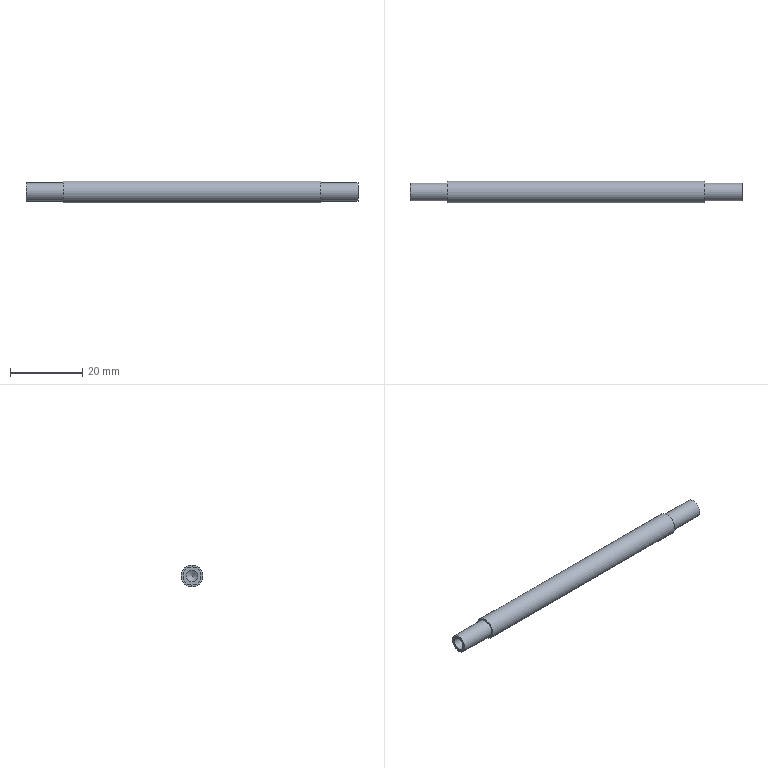Component | NX | WHEEL_AXLE | 1 solid | 11 faces | box 91.6 x 6 x 6 mm | volume 2235 mm3 | cylinder 5 | plane 4 | cone 2 | commonest cylinder face diameters 5 x2 3.3 x2 6 x1
STEP:
#1=CARTESIAN_POINT('',(0.,0.,0.));
#2=DIRECTION('',(0.,0.,1.));
#3=DIRECTION('',(1.,0.,0.));
#4=AXIS2_PLACEMENT_3D('',#1,#2,#3);
#5=CARTESIAN_POINT('',(-49.856,16.19,-74.915));
#6=VERTEX_POINT('',#5);
#7=CARTESIAN_POINT('',(-49.856,16.19,-77.415));
#8=DIRECTION('',(-1.,0.,0.));
#9=DIRECTION('',(0.,0.,1.));
#10=AXIS2_PLACEMENT_3D('',#7,#8,#9);
#11=CIRCLE('',#10,2.5);
#12=CARTESIAN_POINT('',(-60.156,16.19,-77.415));
#13=DIRECTION('',(1.,0.,0.));
#14=DIRECTION('',(0.,0.,-1.));
#15=AXIS2_PLACEMENT_3D('',#12,#13,#14);
#16=CYLINDRICAL_SURFACE('',#15,2.5);
#17=CARTESIAN_POINT('',(9.425,10.3));
#18=DIRECTION('',(-1.,0.));
#19=VECTOR('',#18,1.);
#20=LINE('',#17,#19);
#21=(GEOMETRIC_REPRESENTATION_CONTEXT(2)PARAMETRIC_REPRESENTATION_CONTEXT()REPRESENTATION_CONTEXT('',''));
#22=DEFINITIONAL_REPRESENTATION('',(#20),#21);
#23=PCURVE('',#16,#22);
#24=CARTESIAN_POINT('',(-49.856,16.19,-77.415));
#25=DIRECTION('',(-1.,0.,0.));
#26=DIRECTION('',(0.,0.,1.));
#27=AXIS2_PLACEMENT_3D('',#24,#25,#26);
#28=PLANE('',#27);
#29=CARTESIAN_POINT('',(0.,0.));
#30=DIRECTION('',(1.,0.));
#31=AXIS2_PLACEMENT_2D('',#29,#30);
#32=CIRCLE('',#31,2.5);
#33=(GEOMETRIC_REPRESENTATION_CONTEXT(2)PARAMETRIC_REPRESENTATION_CONTEXT()REPRESENTATION_CONTEXT('',''));
#34=DEFINITIONAL_REPRESENTATION('',(#32),#33);
#35=PCURVE('',#28,#34);
#36=SURFACE_CURVE('',#11,(#23,#35),.PCURVE_S1.);
#37=EDGE_CURVE('',#6,#6,#36,.T.);
#38=ORIENTED_EDGE('',*,*,#37,.T.);
#39=CARTESIAN_POINT('',(-60.156,16.19,-74.915));
#40=VERTEX_POINT('',#39);
#41=CARTESIAN_POINT('',(-60.156,16.19,-74.915));
#42=CARTESIAN_POINT('',(-49.856,16.19,-74.915));
#43=B_SPLINE_CURVE_WITH_KNOTS('',1,(#41,#42),.UNSPECIFIED.,.F.,.F.,(2,2),(0.,10.3),.PIECEWISE_BEZIER_KNOTS.);
#44=CARTESIAN_POINT('',(3.142,0.));
#45=DIRECTION('',(0.,1.));
#46=VECTOR('',#45,1.);
#47=LINE('',#44,#46);
#48=(GEOMETRIC_REPRESENTATION_CONTEXT(2)PARAMETRIC_REPRESENTATION_CONTEXT()REPRESENTATION_CONTEXT('',''));
#49=DEFINITIONAL_REPRESENTATION('',(#47),#48);
#50=PCURVE('',#16,#49);
#51=CARTESIAN_POINT('',(9.425,0.));
#52=DIRECTION('',(0.,1.));
#53=VECTOR('',#52,1.);
#54=LINE('',#51,#53);
#55=(GEOMETRIC_REPRESENTATION_CONTEXT(2)PARAMETRIC_REPRESENTATION_CONTEXT()REPRESENTATION_CONTEXT('',''));
#56=DEFINITIONAL_REPRESENTATION('',(#54),#55);
#57=PCURVE('',#16,#56);
#58=SEAM_CURVE('',#43,(#50,#57),.PCURVE_S1.);
#59=EDGE_CURVE('',#40,#6,#58,.T.);
#60=ORIENTED_EDGE('',*,*,#59,.F.);
#61=CARTESIAN_POINT('',(-60.156,16.19,-77.415));
#62=DIRECTION('',(-1.,0.,0.));
#63=DIRECTION('',(0.,0.,1.));
#64=AXIS2_PLACEMENT_3D('',#61,#62,#63);
#65=CIRCLE('',#64,2.5);
#66=CARTESIAN_POINT('',(9.425,0.));
#67=DIRECTION('',(-1.,0.));
#68=VECTOR('',#67,1.);
#69=LINE('',#66,#68);
#70=(GEOMETRIC_REPRESENTATION_CONTEXT(2)PARAMETRIC_REPRESENTATION_CONTEXT()REPRESENTATION_CONTEXT('',''));
#71=DEFINITIONAL_REPRESENTATION('',(#69),#70);
#72=PCURVE('',#16,#71);
#73=CARTESIAN_POINT('',(-60.156,16.19,-77.415));
#74=DIRECTION('',(-1.,0.,0.));
#75=DIRECTION('',(0.,0.,1.));
#76=AXIS2_PLACEMENT_3D('',#73,#74,#75);
#77=PLANE('',#76);
#78=CARTESIAN_POINT('',(0.,0.));
#79=DIRECTION('',(1.,0.));
#80=AXIS2_PLACEMENT_2D('',#78,#79);
#81=CIRCLE('',#80,2.5);
#82=(GEOMETRIC_REPRESENTATION_CONTEXT(2)PARAMETRIC_REPRESENTATION_CONTEXT()REPRESENTATION_CONTEXT('',''));
#83=DEFINITIONAL_REPRESENTATION('',(#81),#82);
#84=PCURVE('',#77,#83);
#85=SURFACE_CURVE('',#65,(#72,#84),.PCURVE_S1.);
#86=EDGE_CURVE('',#40,#40,#85,.T.);
#87=ORIENTED_EDGE('',*,*,#86,.F.);
#88=ORIENTED_EDGE('',*,*,#59,.T.);
#89=EDGE_LOOP('',(#38,#60,#87,#88));
#90=FACE_BOUND('',#89,.T.);
#91=ADVANCED_FACE('',(#90),#16,.T.);
#92=CARTESIAN_POINT('',(-60.156,16.19,-79.065));
#93=VERTEX_POINT('',#92);
#94=CARTESIAN_POINT('',(-60.156,16.19,-77.415));
#95=DIRECTION('',(1.,0.,0.));
#96=DIRECTION('',(0.,0.,-1.));
#97=AXIS2_PLACEMENT_3D('',#94,#95,#96);
#98=CIRCLE('',#97,1.65);
#99=CARTESIAN_POINT('',(-1.65,0.));
#100=CARTESIAN_POINT('',(-1.65,2.858));
#101=CARTESIAN_POINT('',(0.825,1.429));
#102=CARTESIAN_POINT('',(3.3,0.));
#103=CARTESIAN_POINT('',(0.825,-1.429));
#104=CARTESIAN_POINT('',(-1.65,-2.858));
#105=CARTESIAN_POINT('',(-1.65,0.));
#106=(BOUNDED_CURVE()B_SPLINE_CURVE(2,(#99,#100,#101,#102,#103,#104,#105),.UNSPECIFIED.,.T.,.F.)B_SPLINE_CURVE_WITH_KNOTS((1,2,2,2,2,1),(-2.094,0.,2.094,4.189,6.283,8.378),.UNSPECIFIED.)CURVE()GEOMETRIC_REPRESENTATION_ITEM()RATIONAL_B_SPLINE_CURVE((1.,0.5,1.,0.5,1.,0.5,1.))REPRESENTATION_ITEM(''));
#107=(GEOMETRIC_REPRESENTATION_CONTEXT(2)PARAMETRIC_REPRESENTATION_CONTEXT()REPRESENTATION_CONTEXT('',''));
#108=DEFINITIONAL_REPRESENTATION('',(#106),#107);
#109=PCURVE('',#77,#108);
#110=CARTESIAN_POINT('',(-60.156,16.19,-77.415));
#111=DIRECTION('',(1.,0.,0.));
#112=DIRECTION('',(0.,0.,-1.));
#113=AXIS2_PLACEMENT_3D('',#110,#111,#112);
#114=CYLINDRICAL_SURFACE('',#113,1.65);
#115=CARTESIAN_POINT('',(0.,0.));
#116=DIRECTION('',(1.,0.));
#117=VECTOR('',#116,1.);
#118=LINE('',#115,#117);
#119=(GEOMETRIC_REPRESENTATION_CONTEXT(2)PARAMETRIC_REPRESENTATION_CONTEXT()REPRESENTATION_CONTEXT('',''));
#120=DEFINITIONAL_REPRESENTATION('',(#118),#119);
#121=PCURVE('',#114,#120);
#122=SURFACE_CURVE('',#98,(#109,#121),.PCURVE_S1.);
#123=EDGE_CURVE('',#93,#93,#122,.T.);
#124=ORIENTED_EDGE('',*,*,#123,.T.);
#125=EDGE_LOOP('',(#124));
#126=FACE_BOUND('',#125,.T.);
#127=ORIENTED_EDGE('',*,*,#86,.T.);
#128=EDGE_LOOP('',(#127));
#129=FACE_BOUND('',#128,.T.);
#130=ADVANCED_FACE('',(#126,#129),#77,.T.);
#131=CARTESIAN_POINT('',(-49.856,16.19,-74.415));
#132=VERTEX_POINT('',#131);
#133=CARTESIAN_POINT('',(-49.856,16.19,-77.415));
#134=DIRECTION('',(-1.,0.,0.));
#135=DIRECTION('',(0.,0.,1.));
#136=AXIS2_PLACEMENT_3D('',#133,#134,#135);
#137=CIRCLE('',#136,3.);
#138=CARTESIAN_POINT('',(-49.856,16.19,-77.415));
#139=DIRECTION('',(1.,0.,0.));
#140=DIRECTION('',(0.,0.,-1.));
#141=AXIS2_PLACEMENT_3D('',#138,#139,#140);
#142=CYLINDRICAL_SURFACE('',#141,3.);
#143=CARTESIAN_POINT('',(9.425,0.));
#144=DIRECTION('',(-1.,0.));
#145=VECTOR('',#144,1.);
#146=LINE('',#143,#145);
#147=(GEOMETRIC_REPRESENTATION_CONTEXT(2)PARAMETRIC_REPRESENTATION_CONTEXT()REPRESENTATION_CONTEXT('',''));
#148=DEFINITIONAL_REPRESENTATION('',(#146),#147);
#149=PCURVE('',#142,#148);
#150=CARTESIAN_POINT('',(0.,0.));
#151=DIRECTION('',(1.,0.));
#152=AXIS2_PLACEMENT_2D('',#150,#151);
#153=CIRCLE('',#152,3.);
#154=(GEOMETRIC_REPRESENTATION_CONTEXT(2)PARAMETRIC_REPRESENTATION_CONTEXT()REPRESENTATION_CONTEXT('',''));
#155=DEFINITIONAL_REPRESENTATION('',(#153),#154);
#156=PCURVE('',#28,#155);
#157=SURFACE_CURVE('',#137,(#149,#156),.PCURVE_S1.);
#158=EDGE_CURVE('',#132,#132,#157,.T.);
#159=ORIENTED_EDGE('',*,*,#158,.F.);
#160=CARTESIAN_POINT('',(21.144,16.19,-74.415));
#161=VERTEX_POINT('',#160);
#162=CARTESIAN_POINT('',(-49.856,16.19,-74.415));
#163=CARTESIAN_POINT('',(21.144,16.19,-74.415));
#164=B_SPLINE_CURVE_WITH_KNOTS('',1,(#162,#163),.UNSPECIFIED.,.F.,.F.,(2,2),(0.,71.),.PIECEWISE_BEZIER_KNOTS.);
#165=CARTESIAN_POINT('',(9.425,0.));
#166=DIRECTION('',(0.,1.));
#167=VECTOR('',#166,1.);
#168=LINE('',#165,#167);
#169=(GEOMETRIC_REPRESENTATION_CONTEXT(2)PARAMETRIC_REPRESENTATION_CONTEXT()REPRESENTATION_CONTEXT('',''));
#170=DEFINITIONAL_REPRESENTATION('',(#168),#169);
#171=PCURVE('',#142,#170);
#172=CARTESIAN_POINT('',(3.142,0.));
#173=DIRECTION('',(0.,1.));
#174=VECTOR('',#173,1.);
#175=LINE('',#172,#174);
#176=(GEOMETRIC_REPRESENTATION_CONTEXT(2)PARAMETRIC_REPRESENTATION_CONTEXT()REPRESENTATION_CONTEXT('',''));
#177=DEFINITIONAL_REPRESENTATION('',(#175),#176);
#178=PCURVE('',#142,#177);
#179=SEAM_CURVE('',#164,(#171,#178),.PCURVE_S1.);
#180=EDGE_CURVE('',#132,#161,#179,.T.);
#181=ORIENTED_EDGE('',*,*,#180,.T.);
#182=CARTESIAN_POINT('',(21.144,16.19,-77.415));
#183=DIRECTION('',(-1.,0.,0.));
#184=DIRECTION('',(0.,0.,1.));
#185=AXIS2_PLACEMENT_3D('',#182,#183,#184);
#186=CIRCLE('',#185,3.);
#187=CARTESIAN_POINT('',(9.425,71.));
#188=DIRECTION('',(-1.,0.));
#189=VECTOR('',#188,1.);
#190=LINE('',#187,#189);
#191=(GEOMETRIC_REPRESENTATION_CONTEXT(2)PARAMETRIC_REPRESENTATION_CONTEXT()REPRESENTATION_CONTEXT('',''));
#192=DEFINITIONAL_REPRESENTATION('',(#190),#191);
#193=PCURVE('',#142,#192);
#194=CARTESIAN_POINT('',(21.144,16.19,-77.415));
#195=DIRECTION('',(-1.,0.,0.));
#196=DIRECTION('',(0.,0.,1.));
#197=AXIS2_PLACEMENT_3D('',#194,#195,#196);
#198=PLANE('',#197);
#199=CARTESIAN_POINT('',(0.,0.));
#200=DIRECTION('',(1.,0.));
#201=AXIS2_PLACEMENT_2D('',#199,#200);
#202=CIRCLE('',#201,3.);
#203=(GEOMETRIC_REPRESENTATION_CONTEXT(2)PARAMETRIC_REPRESENTATION_CONTEXT()REPRESENTATION_CONTEXT('',''));
#204=DEFINITIONAL_REPRESENTATION('',(#202),#203);
#205=PCURVE('',#198,#204);
#206=SURFACE_CURVE('',#186,(#193,#205),.PCURVE_S1.);
#207=EDGE_CURVE('',#161,#161,#206,.T.);
#208=ORIENTED_EDGE('',*,*,#207,.T.);
#209=ORIENTED_EDGE('',*,*,#180,.F.);
#210=EDGE_LOOP('',(#159,#181,#208,#209));
#211=FACE_BOUND('',#210,.T.);
#212=ADVANCED_FACE('',(#211),#142,.T.);
#213=ORIENTED_EDGE('',*,*,#37,.F.);
#214=EDGE_LOOP('',(#213));
#215=FACE_BOUND('',#214,.T.);
#216=ORIENTED_EDGE('',*,*,#158,.T.);
#217=EDGE_LOOP('',(#216));
#218=FACE_BOUND('',#217,.T.);
#219=ADVANCED_FACE('',(#215,#218),#28,.T.);
#220=CARTESIAN_POINT('',(21.144,16.19,-74.915));
#221=VERTEX_POINT('',#220);
#222=CARTESIAN_POINT('',(21.144,16.19,-77.415));
#223=DIRECTION('',(-1.,0.,0.));
#224=DIRECTION('',(0.,0.,1.));
#225=AXIS2_PLACEMENT_3D('',#222,#223,#224);
#226=CIRCLE('',#225,2.5);
#227=CARTESIAN_POINT('',(0.,0.));
#228=DIRECTION('',(1.,0.));
#229=AXIS2_PLACEMENT_2D('',#227,#228);
#230=CIRCLE('',#229,2.5);
#231=(GEOMETRIC_REPRESENTATION_CONTEXT(2)PARAMETRIC_REPRESENTATION_CONTEXT()REPRESENTATION_CONTEXT('',''));
#232=DEFINITIONAL_REPRESENTATION('',(#230),#231);
#233=PCURVE('',#198,#232);
#234=CARTESIAN_POINT('',(-60.156,16.19,-77.415));
#235=DIRECTION('',(1.,0.,0.));
#236=DIRECTION('',(0.,0.,-1.));
#237=AXIS2_PLACEMENT_3D('',#234,#235,#236);
#238=CYLINDRICAL_SURFACE('',#237,2.5);
#239=CARTESIAN_POINT('',(9.425,81.3));
#240=DIRECTION('',(-1.,0.));
#241=VECTOR('',#240,1.);
#242=LINE('',#239,#241);
#243=(GEOMETRIC_REPRESENTATION_CONTEXT(2)PARAMETRIC_REPRESENTATION_CONTEXT()REPRESENTATION_CONTEXT('',''));
#244=DEFINITIONAL_REPRESENTATION('',(#242),#243);
#245=PCURVE('',#238,#244);
#246=SURFACE_CURVE('',#226,(#233,#245),.PCURVE_S1.);
#247=EDGE_CURVE('',#221,#221,#246,.T.);
#248=ORIENTED_EDGE('',*,*,#247,.T.);
#249=EDGE_LOOP('',(#248));
#250=FACE_BOUND('',#249,.T.);
#251=ORIENTED_EDGE('',*,*,#207,.F.);
#252=EDGE_LOOP('',(#251));
#253=FACE_BOUND('',#252,.T.);
#254=ADVANCED_FACE('',(#250,#253),#198,.F.);
#255=CARTESIAN_POINT('',(31.444,16.19,-75.765));
#256=VERTEX_POINT('',#255);
#257=CARTESIAN_POINT('',(31.444,16.19,-77.415));
#258=DIRECTION('',(-1.,0.,0.));
#259=DIRECTION('',(0.,0.,1.));
#260=AXIS2_PLACEMENT_3D('',#257,#258,#259);
#261=CIRCLE('',#260,1.65);
#262=CARTESIAN_POINT('',(31.444,16.19,-77.415));
#263=DIRECTION('',(-1.,0.,0.));
#264=DIRECTION('',(0.,0.,1.));
#265=AXIS2_PLACEMENT_3D('',#262,#263,#264);
#266=PLANE('',#265);
#267=CARTESIAN_POINT('',(0.,0.));
#268=DIRECTION('',(1.,0.));
#269=AXIS2_PLACEMENT_2D('',#267,#268);
#270=CIRCLE('',#269,1.65);
#271=(GEOMETRIC_REPRESENTATION_CONTEXT(2)PARAMETRIC_REPRESENTATION_CONTEXT()REPRESENTATION_CONTEXT('',''));
#272=DEFINITIONAL_REPRESENTATION('',(#270),#271);
#273=PCURVE('',#266,#272);
#274=CARTESIAN_POINT('',(31.444,16.19,-77.415));
#275=DIRECTION('',(-1.,0.,0.));
#276=DIRECTION('',(0.,0.,1.));
#277=AXIS2_PLACEMENT_3D('',#274,#275,#276);
#278=CYLINDRICAL_SURFACE('',#277,1.65);
#279=CARTESIAN_POINT('',(0.,0.));
#280=DIRECTION('',(1.,0.));
#281=VECTOR('',#280,1.);
#282=LINE('',#279,#281);
#283=(GEOMETRIC_REPRESENTATION_CONTEXT(2)PARAMETRIC_REPRESENTATION_CONTEXT()REPRESENTATION_CONTEXT('',''));
#284=DEFINITIONAL_REPRESENTATION('',(#282),#283);
#285=PCURVE('',#278,#284);
#286=SURFACE_CURVE('',#261,(#273,#285),.PCURVE_S1.);
#287=EDGE_CURVE('',#256,#256,#286,.T.);
#288=ORIENTED_EDGE('',*,*,#287,.T.);
#289=EDGE_LOOP('',(#288));
#290=FACE_BOUND('',#289,.T.);
#291=CARTESIAN_POINT('',(31.444,16.19,-74.915));
#292=VERTEX_POINT('',#291);
#293=CARTESIAN_POINT('',(31.444,16.19,-77.415));
#294=DIRECTION('',(-1.,0.,0.));
#295=DIRECTION('',(0.,0.,1.));
#296=AXIS2_PLACEMENT_3D('',#293,#294,#295);
#297=CIRCLE('',#296,2.5);
#298=CARTESIAN_POINT('',(0.,0.));
#299=DIRECTION('',(1.,0.));
#300=AXIS2_PLACEMENT_2D('',#298,#299);
#301=CIRCLE('',#300,2.5);
#302=(GEOMETRIC_REPRESENTATION_CONTEXT(2)PARAMETRIC_REPRESENTATION_CONTEXT()REPRESENTATION_CONTEXT('',''));
#303=DEFINITIONAL_REPRESENTATION('',(#301),#302);
#304=PCURVE('',#266,#303);
#305=CARTESIAN_POINT('',(9.425,91.6));
#306=DIRECTION('',(-1.,0.));
#307=VECTOR('',#306,1.);
#308=LINE('',#305,#307);
#309=(GEOMETRIC_REPRESENTATION_CONTEXT(2)PARAMETRIC_REPRESENTATION_CONTEXT()REPRESENTATION_CONTEXT('',''));
#310=DEFINITIONAL_REPRESENTATION('',(#308),#309);
#311=PCURVE('',#238,#310);
#312=SURFACE_CURVE('',#297,(#304,#311),.PCURVE_S1.);
#313=EDGE_CURVE('',#292,#292,#312,.T.);
#314=ORIENTED_EDGE('',*,*,#313,.F.);
#315=EDGE_LOOP('',(#314));
#316=FACE_BOUND('',#315,.T.);
#317=ADVANCED_FACE('',(#290,#316),#266,.F.);
#318=ORIENTED_EDGE('',*,*,#313,.T.);
#319=CARTESIAN_POINT('',(21.144,16.19,-74.915));
#320=CARTESIAN_POINT('',(31.444,16.19,-74.915));
#321=B_SPLINE_CURVE_WITH_KNOTS('',1,(#319,#320),.UNSPECIFIED.,.F.,.F.,(2,2),(81.3,91.6),.PIECEWISE_BEZIER_KNOTS.);
#322=CARTESIAN_POINT('',(3.142,0.));
#323=DIRECTION('',(0.,1.));
#324=VECTOR('',#323,1.);
#325=LINE('',#322,#324);
#326=(GEOMETRIC_REPRESENTATION_CONTEXT(2)PARAMETRIC_REPRESENTATION_CONTEXT()REPRESENTATION_CONTEXT('',''));
#327=DEFINITIONAL_REPRESENTATION('',(#325),#326);
#328=PCURVE('',#238,#327);
#329=CARTESIAN_POINT('',(9.425,0.));
#330=DIRECTION('',(0.,1.));
#331=VECTOR('',#330,1.);
#332=LINE('',#329,#331);
#333=(GEOMETRIC_REPRESENTATION_CONTEXT(2)PARAMETRIC_REPRESENTATION_CONTEXT()REPRESENTATION_CONTEXT('',''));
#334=DEFINITIONAL_REPRESENTATION('',(#332),#333);
#335=PCURVE('',#238,#334);
#336=SEAM_CURVE('',#321,(#328,#335),.PCURVE_S1.);
#337=EDGE_CURVE('',#221,#292,#336,.T.);
#338=ORIENTED_EDGE('',*,*,#337,.F.);
#339=ORIENTED_EDGE('',*,*,#247,.F.);
#340=ORIENTED_EDGE('',*,*,#337,.T.);
#341=EDGE_LOOP('',(#318,#338,#339,#340));
#342=FACE_BOUND('',#341,.T.);
#343=ADVANCED_FACE('',(#342),#238,.T.);
#344=CARTESIAN_POINT('',(-50.156,16.19,-75.765));
#345=VERTEX_POINT('',#344);
#346=CARTESIAN_POINT('',(-50.156,16.19,-79.065));
#347=VERTEX_POINT('',#346);
#348=CARTESIAN_POINT('',(-50.156,16.19,-77.415));
#349=DIRECTION('',(-1.,0.,0.));
#350=DIRECTION('',(0.,0.,-1.));
#351=AXIS2_PLACEMENT_3D('',#348,#349,#350);
#352=CIRCLE('',#351,1.65);
#353=CARTESIAN_POINT('',(-50.156,16.19,-77.415));
#354=DIRECTION('',(-1.,0.,0.));
#355=DIRECTION('',(0.,0.,1.));
#356=AXIS2_PLACEMENT_3D('',#353,#354,#355);
#357=CONICAL_SURFACE('',#356,1.65,1.03);
#358=CARTESIAN_POINT('',(-3.142,0.));
#359=DIRECTION('',(1.,0.));
#360=VECTOR('',#359,1.);
#361=LINE('',#358,#360);
#362=(GEOMETRIC_REPRESENTATION_CONTEXT(2)PARAMETRIC_REPRESENTATION_CONTEXT()REPRESENTATION_CONTEXT('',''));
#363=DEFINITIONAL_REPRESENTATION('',(#361),#362);
#364=PCURVE('',#357,#363);
#365=CARTESIAN_POINT('',(6.283,10.));
#366=DIRECTION('',(-1.,0.));
#367=VECTOR('',#366,1.);
#368=LINE('',#365,#367);
#369=(GEOMETRIC_REPRESENTATION_CONTEXT(2)PARAMETRIC_REPRESENTATION_CONTEXT()REPRESENTATION_CONTEXT('',''));
#370=DEFINITIONAL_REPRESENTATION('',(#368),#369);
#371=PCURVE('',#114,#370);
#372=SURFACE_CURVE('',#352,(#364,#371),.PCURVE_S1.);
#373=EDGE_CURVE('',#345,#347,#372,.T.);
#374=ORIENTED_EDGE('',*,*,#373,.F.);
#375=CARTESIAN_POINT('',(-49.164,16.19,-77.415));
#376=VERTEX_POINT('',#375);
#377=CARTESIAN_POINT('',(-49.164,16.19,-77.415));
#378=CARTESIAN_POINT('',(-50.156,16.19,-75.765));
#379=B_SPLINE_CURVE_WITH_KNOTS('',1,(#377,#378),.UNSPECIFIED.,.F.,.F.,(2,2),(-1.925,0.),.PIECEWISE_BEZIER_KNOTS.);
#380=CARTESIAN_POINT('',(0.,0.));
#381=DIRECTION('',(0.,1.));
#382=VECTOR('',#381,1.);
#383=LINE('',#380,#382);
#384=(GEOMETRIC_REPRESENTATION_CONTEXT(2)PARAMETRIC_REPRESENTATION_CONTEXT()REPRESENTATION_CONTEXT('',''));
#385=DEFINITIONAL_REPRESENTATION('',(#383),#384);
#386=PCURVE('',#357,#385);
#387=CARTESIAN_POINT('',(6.283,0.));
#388=DIRECTION('',(0.,1.));
#389=VECTOR('',#388,1.);
#390=LINE('',#387,#389);
#391=(GEOMETRIC_REPRESENTATION_CONTEXT(2)PARAMETRIC_REPRESENTATION_CONTEXT()REPRESENTATION_CONTEXT('',''));
#392=DEFINITIONAL_REPRESENTATION('',(#390),#391);
#393=PCURVE('',#357,#392);
#394=SEAM_CURVE('',#379,(#386,#393),.PCURVE_S1.);
#395=EDGE_CURVE('',#376,#345,#394,.T.);
#396=ORIENTED_EDGE('',*,*,#395,.F.);
#397=ORIENTED_EDGE('',*,*,#395,.T.);
#398=CARTESIAN_POINT('',(-50.156,16.19,-77.415));
#399=DIRECTION('',(-1.,0.,0.));
#400=DIRECTION('',(0.,0.,-1.));
#401=AXIS2_PLACEMENT_3D('',#398,#399,#400);
#402=CIRCLE('',#401,1.65);
#403=CARTESIAN_POINT('',(3.142,0.));
#404=DIRECTION('',(1.,0.));
#405=VECTOR('',#404,1.);
#406=LINE('',#403,#405);
#407=(GEOMETRIC_REPRESENTATION_CONTEXT(2)PARAMETRIC_REPRESENTATION_CONTEXT()REPRESENTATION_CONTEXT('',''));
#408=DEFINITIONAL_REPRESENTATION('',(#406),#407);
#409=PCURVE('',#357,#408);
#410=CARTESIAN_POINT('',(6.283,10.));
#411=DIRECTION('',(-1.,0.));
#412=VECTOR('',#411,1.);
#413=LINE('',#410,#412);
#414=(GEOMETRIC_REPRESENTATION_CONTEXT(2)PARAMETRIC_REPRESENTATION_CONTEXT()REPRESENTATION_CONTEXT('',''));
#415=DEFINITIONAL_REPRESENTATION('',(#413),#414);
#416=PCURVE('',#114,#415);
#417=SURFACE_CURVE('',#402,(#409,#416),.PCURVE_S1.);
#418=EDGE_CURVE('',#347,#345,#417,.T.);
#419=ORIENTED_EDGE('',*,*,#418,.F.);
#420=EDGE_LOOP('',(#374,#396,#397,#419));
#421=FACE_BOUND('',#420,.F.);
#422=ADVANCED_FACE('',(#421),#357,.F.);
#423=ORIENTED_EDGE('',*,*,#373,.T.);
#424=CARTESIAN_POINT('',(-60.156,16.19,-79.065));
#425=CARTESIAN_POINT('',(-50.156,16.19,-79.065));
#426=B_SPLINE_CURVE_WITH_KNOTS('',1,(#424,#425),.UNSPECIFIED.,.F.,.F.,(2,2),(0.,10.),.PIECEWISE_BEZIER_KNOTS.);
#427=CARTESIAN_POINT('',(0.,0.));
#428=DIRECTION('',(0.,1.));
#429=VECTOR('',#428,1.);
#430=LINE('',#427,#429);
#431=(GEOMETRIC_REPRESENTATION_CONTEXT(2)PARAMETRIC_REPRESENTATION_CONTEXT()REPRESENTATION_CONTEXT('',''));
#432=DEFINITIONAL_REPRESENTATION('',(#430),#431);
#433=PCURVE('',#114,#432);
#434=CARTESIAN_POINT('',(6.283,0.));
#435=DIRECTION('',(0.,1.));
#436=VECTOR('',#435,1.);
#437=LINE('',#434,#436);
#438=(GEOMETRIC_REPRESENTATION_CONTEXT(2)PARAMETRIC_REPRESENTATION_CONTEXT()REPRESENTATION_CONTEXT('',''));
#439=DEFINITIONAL_REPRESENTATION('',(#437),#438);
#440=PCURVE('',#114,#439);
#441=SEAM_CURVE('',#426,(#433,#440),.PCURVE_S1.);
#442=EDGE_CURVE('',#93,#347,#441,.T.);
#443=ORIENTED_EDGE('',*,*,#442,.F.);
#444=ORIENTED_EDGE('',*,*,#123,.T.);
#445=ORIENTED_EDGE('',*,*,#442,.T.);
#446=ORIENTED_EDGE('',*,*,#418,.T.);
#447=EDGE_LOOP('',(#423,#443,#444,#445,#446));
#448=FACE_BOUND('',#447,.F.);
#449=ADVANCED_FACE('',(#448),#114,.F.);
#450=CARTESIAN_POINT('',(21.444,16.19,-79.065));
#451=VERTEX_POINT('',#450);
#452=CARTESIAN_POINT('',(21.444,16.19,-75.765));
#453=VERTEX_POINT('',#452);
#454=CARTESIAN_POINT('',(21.444,16.19,-77.415));
#455=DIRECTION('',(1.,0.,0.));
#456=DIRECTION('',(0.,0.,1.));
#457=AXIS2_PLACEMENT_3D('',#454,#455,#456);
#458=CIRCLE('',#457,1.65);
#459=CARTESIAN_POINT('',(21.444,16.19,-77.415));
#460=DIRECTION('',(1.,0.,0.));
#461=DIRECTION('',(0.,0.,-1.));
#462=AXIS2_PLACEMENT_3D('',#459,#460,#461);
#463=CONICAL_SURFACE('',#462,1.65,1.03);
#464=CARTESIAN_POINT('',(-3.142,0.));
#465=DIRECTION('',(1.,0.));
#466=VECTOR('',#465,1.);
#467=LINE('',#464,#466);
#468=(GEOMETRIC_REPRESENTATION_CONTEXT(2)PARAMETRIC_REPRESENTATION_CONTEXT()REPRESENTATION_CONTEXT('',''));
#469=DEFINITIONAL_REPRESENTATION('',(#467),#468);
#470=PCURVE('',#463,#469);
#471=CARTESIAN_POINT('',(6.283,10.));
#472=DIRECTION('',(-1.,0.));
#473=VECTOR('',#472,1.);
#474=LINE('',#471,#473);
#475=(GEOMETRIC_REPRESENTATION_CONTEXT(2)PARAMETRIC_REPRESENTATION_CONTEXT()REPRESENTATION_CONTEXT('',''));
#476=DEFINITIONAL_REPRESENTATION('',(#474),#475);
#477=PCURVE('',#278,#476);
#478=SURFACE_CURVE('',#458,(#470,#477),.PCURVE_S1.);
#479=EDGE_CURVE('',#451,#453,#478,.T.);
#480=ORIENTED_EDGE('',*,*,#479,.F.);
#481=CARTESIAN_POINT('',(20.453,16.19,-77.415));
#482=VERTEX_POINT('',#481);
#483=CARTESIAN_POINT('',(20.453,16.19,-77.415));
#484=CARTESIAN_POINT('',(21.444,16.19,-79.065));
#485=B_SPLINE_CURVE_WITH_KNOTS('',1,(#483,#484),.UNSPECIFIED.,.F.,.F.,(2,2),(-1.925,0.),.PIECEWISE_BEZIER_KNOTS.);
#486=CARTESIAN_POINT('',(0.,0.));
#487=DIRECTION('',(0.,1.));
#488=VECTOR('',#487,1.);
#489=LINE('',#486,#488);
#490=(GEOMETRIC_REPRESENTATION_CONTEXT(2)PARAMETRIC_REPRESENTATION_CONTEXT()REPRESENTATION_CONTEXT('',''));
#491=DEFINITIONAL_REPRESENTATION('',(#489),#490);
#492=PCURVE('',#463,#491);
#493=CARTESIAN_POINT('',(6.283,0.));
#494=DIRECTION('',(0.,1.));
#495=VECTOR('',#494,1.);
#496=LINE('',#493,#495);
#497=(GEOMETRIC_REPRESENTATION_CONTEXT(2)PARAMETRIC_REPRESENTATION_CONTEXT()REPRESENTATION_CONTEXT('',''));
#498=DEFINITIONAL_REPRESENTATION('',(#496),#497);
#499=PCURVE('',#463,#498);
#500=SEAM_CURVE('',#485,(#492,#499),.PCURVE_S1.);
#501=EDGE_CURVE('',#482,#451,#500,.T.);
#502=ORIENTED_EDGE('',*,*,#501,.F.);
#503=ORIENTED_EDGE('',*,*,#501,.T.);
#504=CARTESIAN_POINT('',(21.444,16.19,-77.415));
#505=DIRECTION('',(1.,0.,0.));
#506=DIRECTION('',(0.,0.,1.));
#507=AXIS2_PLACEMENT_3D('',#504,#505,#506);
#508=CIRCLE('',#507,1.65);
#509=CARTESIAN_POINT('',(3.142,0.));
#510=DIRECTION('',(1.,0.));
#511=VECTOR('',#510,1.);
#512=LINE('',#509,#511);
#513=(GEOMETRIC_REPRESENTATION_CONTEXT(2)PARAMETRIC_REPRESENTATION_CONTEXT()REPRESENTATION_CONTEXT('',''));
#514=DEFINITIONAL_REPRESENTATION('',(#512),#513);
#515=PCURVE('',#463,#514);
#516=CARTESIAN_POINT('',(6.283,10.));
#517=DIRECTION('',(-1.,0.));
#518=VECTOR('',#517,1.);
#519=LINE('',#516,#518);
#520=(GEOMETRIC_REPRESENTATION_CONTEXT(2)PARAMETRIC_REPRESENTATION_CONTEXT()REPRESENTATION_CONTEXT('',''));
#521=DEFINITIONAL_REPRESENTATION('',(#519),#520);
#522=PCURVE('',#278,#521);
#523=SURFACE_CURVE('',#508,(#515,#522),.PCURVE_S1.);
#524=EDGE_CURVE('',#453,#451,#523,.T.);
#525=ORIENTED_EDGE('',*,*,#524,.F.);
#526=EDGE_LOOP('',(#480,#502,#503,#525));
#527=FACE_BOUND('',#526,.F.);
#528=ADVANCED_FACE('',(#527),#463,.F.);
#529=ORIENTED_EDGE('',*,*,#479,.T.);
#530=CARTESIAN_POINT('',(31.444,16.19,-75.765));
#531=CARTESIAN_POINT('',(21.444,16.19,-75.765));
#532=B_SPLINE_CURVE_WITH_KNOTS('',1,(#530,#531),.UNSPECIFIED.,.F.,.F.,(2,2),(0.,10.),.PIECEWISE_BEZIER_KNOTS.);
#533=CARTESIAN_POINT('',(0.,0.));
#534=DIRECTION('',(0.,1.));
#535=VECTOR('',#534,1.);
#536=LINE('',#533,#535);
#537=(GEOMETRIC_REPRESENTATION_CONTEXT(2)PARAMETRIC_REPRESENTATION_CONTEXT()REPRESENTATION_CONTEXT('',''));
#538=DEFINITIONAL_REPRESENTATION('',(#536),#537);
#539=PCURVE('',#278,#538);
#540=CARTESIAN_POINT('',(6.283,0.));
#541=DIRECTION('',(0.,1.));
#542=VECTOR('',#541,1.);
#543=LINE('',#540,#542);
#544=(GEOMETRIC_REPRESENTATION_CONTEXT(2)PARAMETRIC_REPRESENTATION_CONTEXT()REPRESENTATION_CONTEXT('',''));
#545=DEFINITIONAL_REPRESENTATION('',(#543),#544);
#546=PCURVE('',#278,#545);
#547=SEAM_CURVE('',#532,(#539,#546),.PCURVE_S1.);
#548=EDGE_CURVE('',#256,#453,#547,.T.);
#549=ORIENTED_EDGE('',*,*,#548,.F.);
#550=ORIENTED_EDGE('',*,*,#287,.T.);
#551=ORIENTED_EDGE('',*,*,#548,.T.);
#552=ORIENTED_EDGE('',*,*,#524,.T.);
#553=EDGE_LOOP('',(#529,#549,#550,#551,#552));
#554=FACE_BOUND('',#553,.F.);
#555=ADVANCED_FACE('',(#554),#278,.F.);
#556=CLOSED_SHELL('',(#91,#130,#212,#219,#254,#317,#343,#422,#449,#528,#555));
#557=MANIFOLD_SOLID_BREP('',#556);
#558=(LENGTH_UNIT()NAMED_UNIT(*)SI_UNIT(.MILLI.,.METRE.));
#559=UNCERTAINTY_MEASURE_WITH_UNIT(LENGTH_MEASURE(0.00001),#558,'','');
#560=(NAMED_UNIT(*)PLANE_ANGLE_UNIT()SI_UNIT($,.RADIAN.));
#561=(NAMED_UNIT(*)SI_UNIT($,.STERADIAN.)SOLID_ANGLE_UNIT());
#562=(GEOMETRIC_REPRESENTATION_CONTEXT(3)GLOBAL_UNCERTAINTY_ASSIGNED_CONTEXT((#559))GLOBAL_UNIT_ASSIGNED_CONTEXT((#558,#560,#561))REPRESENTATION_CONTEXT('',''));
#563=ADVANCED_BREP_SHAPE_REPRESENTATION('',(#4,#557),#562);